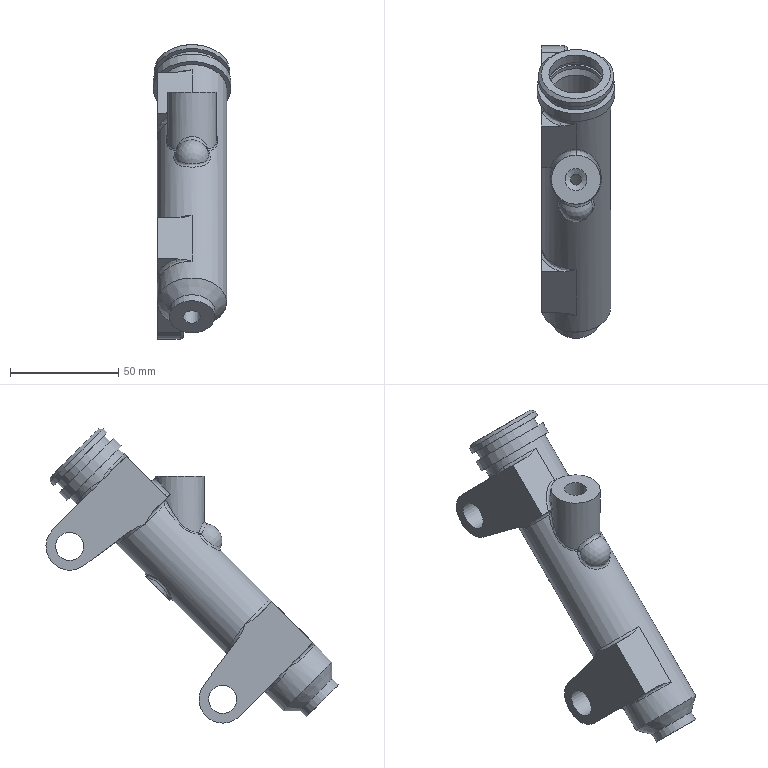Component | NX | WORKPIECE | 1 solid | 88 faces | volume 91704 mm3 | cylinder 28 | plane 25 | spline 19 | torus 8 | cone 5 | sphere 3 | commonest cylinder face diameters 3 x6 22 x3 15.5 x2 4.5 x2 13 x2 25 x2 32 x1 21 x1